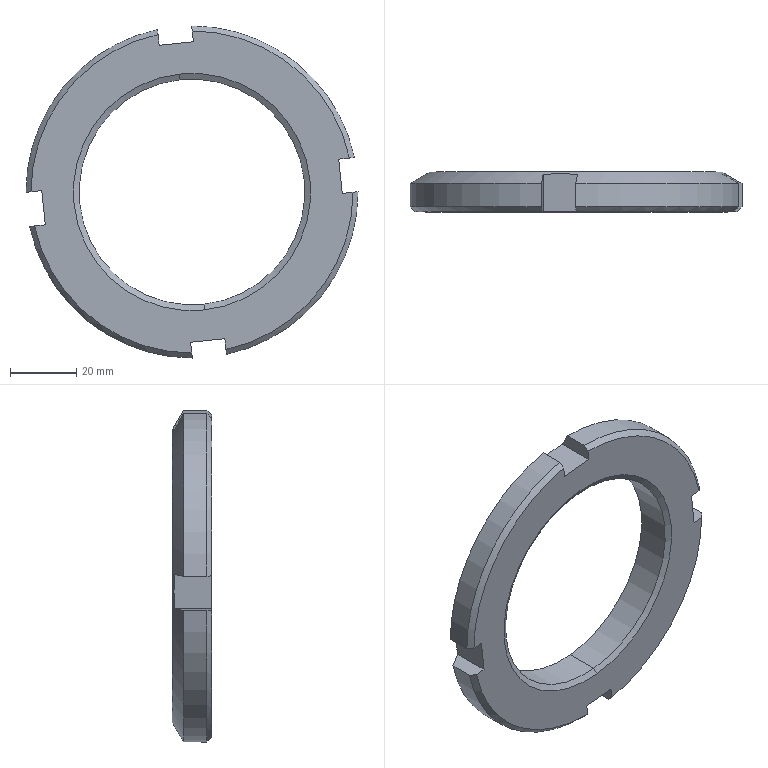Component | SolidWorks | LowerTensioningDeviceAssembly-1_GB_T812-1988[RoundNutM68_2]-1 | 1 solid | 30 faces | box 100 x 12 x 100 mm | volume 44820 mm3 | plane 14 | cone 10 | cylinder 6 | commonest cylinder face diameters 100 x4 68 x2
STEP:
#1=COLOUR_RGB('',0.7922,0.8196,0.9333);
#2=FILL_AREA_STYLE_COLOUR('',#1);
#3=FILL_AREA_STYLE('',(#2));
#4=SURFACE_STYLE_FILL_AREA(#3);
#5=SURFACE_SIDE_STYLE('',(#4));
#6=SURFACE_STYLE_USAGE(.BOTH.,#5);
#7=PRESENTATION_STYLE_ASSIGNMENT((#6));
#8=CARTESIAN_POINT('',(-0.1409,6.654,0.03981));
#9=VERTEX_POINT('',#8);
#10=CARTESIAN_POINT('',(0.1409,6.654,-2.622));
#11=VERTEX_POINT('',#10);
#12=CARTESIAN_POINT('',(-0.,6.654,-1.291));
#13=DIRECTION('',(-0.,-1.,-0.));
#14=DIRECTION('',(0.1053,0.,-0.9944));
#15=AXIS2_PLACEMENT_3D('',#12,#13,#14);
#16=CIRCLE('',#15,1.339);
#17=EDGE_CURVE('',#9,#11,#16,.T.);
#18=ORIENTED_EDGE('',*,*,#17,.F.);
#19=CARTESIAN_POINT('',(-0.1481,6.614,0.1076));
#20=VERTEX_POINT('',#19);
#21=CARTESIAN_POINT('',(-0.1409,6.654,0.03981));
#22=DIRECTION('',(-0.09115,-0.5,0.8612));
#23=VECTOR('',#22,39.37);
#24=LINE('',#21,#23);
#25=EDGE_CURVE('',#9,#20,#24,.T.);
#26=ORIENTED_EDGE('',*,*,#25,.T.);
#27=CARTESIAN_POINT('',(0.1481,6.614,-2.69));
#28=VERTEX_POINT('',#27);
#29=CARTESIAN_POINT('',(-0.,6.614,-1.291));
#30=DIRECTION('',(0.,1.,0.));
#31=DIRECTION('',(0.1053,0.,-0.9944));
#32=AXIS2_PLACEMENT_3D('',#29,#30,#31);
#33=CIRCLE('',#32,1.407);
#34=EDGE_CURVE('',#28,#20,#33,.T.);
#35=ORIENTED_EDGE('',*,*,#34,.F.);
#36=CARTESIAN_POINT('',(0.1409,6.654,-2.622));
#37=DIRECTION('',(0.09115,-0.5,-0.8612));
#38=VECTOR('',#37,39.37);
#39=LINE('',#36,#38);
#40=EDGE_CURVE('',#11,#28,#39,.T.);
#41=ORIENTED_EDGE('',*,*,#40,.F.);
#42=EDGE_LOOP('',(#18,#26,#35,#41));
#43=FACE_OUTER_BOUND('',#42,.T.);
#44=CARTESIAN_POINT('',(-0.,6.654,-1.291));
#45=DIRECTION('',(-0.,-1.,-0.));
#46=DIRECTION('',(0.1053,0.,-0.9944));
#47=AXIS2_PLACEMENT_3D('',#44,#45,#46);
#48=CONICAL_SURFACE('',#47,1.339,1.047);
#49=ADVANCED_FACE('',(#43),#48,.F.);
#50=CARTESIAN_POINT('',(0.1409,7.047,-2.622));
#51=VERTEX_POINT('',#50);
#52=CARTESIAN_POINT('',(-0.1409,7.047,0.03981));
#53=VERTEX_POINT('',#52);
#54=CARTESIAN_POINT('',(-0.,7.047,-1.291));
#55=DIRECTION('',(0.,1.,0.));
#56=DIRECTION('',(0.1053,0.,-0.9944));
#57=AXIS2_PLACEMENT_3D('',#54,#55,#56);
#58=CIRCLE('',#57,1.339);
#59=EDGE_CURVE('',#51,#53,#58,.T.);
#60=ORIENTED_EDGE('',*,*,#59,.F.);
#61=CARTESIAN_POINT('',(0.1481,7.087,-2.69));
#62=VERTEX_POINT('',#61);
#63=CARTESIAN_POINT('',(0.1481,7.087,-2.69));
#64=DIRECTION('',(0.09115,0.5,-0.8612));
#65=VECTOR('',#64,39.37);
#66=LINE('',#63,#65);
#67=EDGE_CURVE('',#51,#62,#66,.T.);
#68=ORIENTED_EDGE('',*,*,#67,.T.);
#69=CARTESIAN_POINT('',(-0.1481,7.087,0.1076));
#70=VERTEX_POINT('',#69);
#71=CARTESIAN_POINT('',(-0.,7.087,-1.291));
#72=DIRECTION('',(-0.,-1.,-0.));
#73=DIRECTION('',(0.1053,0.,-0.9944));
#74=AXIS2_PLACEMENT_3D('',#71,#72,#73);
#75=CIRCLE('',#74,1.407);
#76=EDGE_CURVE('',#70,#62,#75,.T.);
#77=ORIENTED_EDGE('',*,*,#76,.F.);
#78=CARTESIAN_POINT('',(-0.1481,7.087,0.1076));
#79=DIRECTION('',(-0.09115,0.5,0.8612));
#80=VECTOR('',#79,39.37);
#81=LINE('',#78,#80);
#82=EDGE_CURVE('',#53,#70,#81,.T.);
#83=ORIENTED_EDGE('',*,*,#82,.F.);
#84=EDGE_LOOP('',(#60,#68,#77,#83));
#85=FACE_OUTER_BOUND('',#84,.T.);
#86=CARTESIAN_POINT('',(-0.,7.087,-1.291));
#87=DIRECTION('',(0.,1.,0.));
#88=DIRECTION('',(-0.1053,-0.,0.9944));
#89=AXIS2_PLACEMENT_3D('',#86,#87,#88);
#90=CONICAL_SURFACE('',#89,1.407,1.047);
#91=ADVANCED_FACE('',(#85),#90,.F.);
#92=CARTESIAN_POINT('',(-0.1823,7.087,0.4313));
#93=VERTEX_POINT('',#92);
#94=CARTESIAN_POINT('',(0.1823,7.087,-3.014));
#95=VERTEX_POINT('',#94);
#96=CARTESIAN_POINT('',(-0.,7.087,-1.291));
#97=DIRECTION('',(0.,1.,0.));
#98=DIRECTION('',(0.1053,0.,-0.9944));
#99=AXIS2_PLACEMENT_3D('',#96,#97,#98);
#100=CIRCLE('',#99,1.732);
#101=EDGE_CURVE('',#93,#95,#100,.T.);
#102=ORIENTED_EDGE('',*,*,#101,.F.);
#103=CARTESIAN_POINT('',(-0.1864,7.064,0.4697));
#104=VERTEX_POINT('',#103);
#105=CARTESIAN_POINT('',(-0.2072,6.95,0.6662));
#106=DIRECTION('',(-0.09115,-0.5,0.8612));
#107=VECTOR('',#106,39.37);
#108=LINE('',#105,#107);
#109=EDGE_CURVE('',#93,#104,#108,.T.);
#110=ORIENTED_EDGE('',*,*,#109,.T.);
#111=CARTESIAN_POINT('',(0.01641,7.058,0.4912));
#112=VERTEX_POINT('',#111);
#113=CARTESIAN_POINT('',(0.01641,7.058,0.4912));
#114=CARTESIAN_POINT('',(-0.051,7.062,0.4841));
#115=CARTESIAN_POINT('',(-0.1186,7.064,0.4769));
#116=CARTESIAN_POINT('',(-0.1864,7.064,0.4697));
#117=B_SPLINE_CURVE_WITH_KNOTS('',3,(#113,#114,#115,#116),.UNSPECIFIED.,.F.,.F.,(4,4),(0.01245,0.01763),.UNSPECIFIED.);
#118=EDGE_CURVE('',#112,#104,#117,.T.);
#119=ORIENTED_EDGE('',*,*,#118,.F.);
#120=CARTESIAN_POINT('',(-0.003271,6.95,0.6772));
#121=VERTEX_POINT('',#120);
#122=CARTESIAN_POINT('',(-0.003271,6.95,0.6772));
#123=CARTESIAN_POINT('',(-0.002137,6.956,0.6665));
#124=CARTESIAN_POINT('',(-0.001004,6.963,0.6557));
#125=CARTESIAN_POINT('',(0.0001294,6.969,0.645));
#126=CARTESIAN_POINT('',(0.005556,6.998,0.5938));
#127=CARTESIAN_POINT('',(0.01098,7.028,0.5425));
#128=CARTESIAN_POINT('',(0.01641,7.058,0.4912));
#129=B_SPLINE_CURVE_WITH_KNOTS('',3,(#122,#123,#124,#125,#126,#127,#128),.UNSPECIFIED.,.F.,.F.,(4,3,4),(0.01027,0.01122,0.01575),.UNSPECIFIED.);
#130=EDGE_CURVE('',#121,#112,#129,.T.);
#131=ORIENTED_EDGE('',*,*,#130,.F.);
#132=CARTESIAN_POINT('',(1.926,6.95,-0.8825));
#133=VERTEX_POINT('',#132);
#134=CARTESIAN_POINT('',(-0.,6.95,-1.291));
#135=DIRECTION('',(-0.,-1.,-0.));
#136=DIRECTION('',(0.1053,0.,-0.9944));
#137=AXIS2_PLACEMENT_3D('',#134,#135,#136);
#138=CIRCLE('',#137,1.969);
#139=EDGE_CURVE('',#133,#121,#138,.T.);
#140=ORIENTED_EDGE('',*,*,#139,.F.);
#141=CARTESIAN_POINT('',(1.74,7.058,-0.9021));
#142=VERTEX_POINT('',#141);
#143=CARTESIAN_POINT('',(1.74,7.058,-0.9021));
#144=CARTESIAN_POINT('',(1.802,7.022,-0.8956));
#145=CARTESIAN_POINT('',(1.864,6.986,-0.889));
#146=CARTESIAN_POINT('',(1.926,6.95,-0.8825));
#147=B_SPLINE_CURVE_WITH_KNOTS('',3,(#143,#144,#145,#146),.UNSPECIFIED.,.F.,.F.,(4,4),(0.01064,0.01612),.UNSPECIFIED.);
#148=EDGE_CURVE('',#142,#133,#147,.T.);
#149=ORIENTED_EDGE('',*,*,#148,.F.);
#150=CARTESIAN_POINT('',(1.783,7.058,-1.308));
#151=VERTEX_POINT('',#150);
#152=CARTESIAN_POINT('',(1.783,7.058,-1.308));
#153=CARTESIAN_POINT('',(1.775,7.062,-1.241));
#154=CARTESIAN_POINT('',(1.768,7.064,-1.173));
#155=CARTESIAN_POINT('',(1.758,7.064,-1.072));
#156=CARTESIAN_POINT('',(1.754,7.064,-1.038));
#157=CARTESIAN_POINT('',(1.747,7.062,-0.97));
#158=CARTESIAN_POINT('',(1.743,7.06,-0.936));
#159=CARTESIAN_POINT('',(1.74,7.058,-0.9021));
#160=B_SPLINE_CURVE_WITH_KNOTS('',3,(#152,#153,#154,#155,#156,#157,#158,#159),.UNSPECIFIED.,.F.,.F.,(4,2,2,4),(0.01245,0.01761,0.02019,0.02278),.UNSPECIFIED.);
#161=EDGE_CURVE('',#151,#142,#160,.T.);
#162=ORIENTED_EDGE('',*,*,#161,.F.);
#163=CARTESIAN_POINT('',(1.969,6.95,-1.288));
#164=VERTEX_POINT('',#163);
#165=CARTESIAN_POINT('',(1.969,6.95,-1.288));
#166=CARTESIAN_POINT('',(1.907,6.986,-1.295));
#167=CARTESIAN_POINT('',(1.845,7.022,-1.301));
#168=CARTESIAN_POINT('',(1.783,7.058,-1.308));
#169=B_SPLINE_CURVE_WITH_KNOTS('',3,(#165,#166,#167,#168),.UNSPECIFIED.,.F.,.F.,(4,4),(0.006321,0.0118),.UNSPECIFIED.);
#170=EDGE_CURVE('',#164,#151,#169,.T.);
#171=ORIENTED_EDGE('',*,*,#170,.F.);
#172=CARTESIAN_POINT('',(0.4089,6.95,-3.217));
#173=VERTEX_POINT('',#172);
#174=CARTESIAN_POINT('',(-0.,6.95,-1.291));
#175=DIRECTION('',(-0.,-1.,-0.));
#176=DIRECTION('',(0.1053,0.,-0.9944));
#177=AXIS2_PLACEMENT_3D('',#174,#175,#176);
#178=CIRCLE('',#177,1.969);
#179=EDGE_CURVE('',#173,#164,#178,.T.);
#180=ORIENTED_EDGE('',*,*,#179,.F.);
#181=CARTESIAN_POINT('',(0.3892,7.058,-3.031));
#182=VERTEX_POINT('',#181);
#183=CARTESIAN_POINT('',(0.3892,7.058,-3.031));
#184=CARTESIAN_POINT('',(0.3958,7.022,-3.093));
#185=CARTESIAN_POINT('',(0.4023,6.986,-3.155));
#186=CARTESIAN_POINT('',(0.4089,6.95,-3.217));
#187=B_SPLINE_CURVE_WITH_KNOTS('',3,(#183,#184,#185,#186),.UNSPECIFIED.,.F.,.F.,(4,4),(0.01064,0.01612),.UNSPECIFIED.);
#188=EDGE_CURVE('',#182,#173,#187,.T.);
#189=ORIENTED_EDGE('',*,*,#188,.F.);
#190=CARTESIAN_POINT('',(0.1864,7.064,-3.052));
#191=VERTEX_POINT('',#190);
#192=CARTESIAN_POINT('',(0.1864,7.064,-3.052));
#193=CARTESIAN_POINT('',(0.2542,7.064,-3.045));
#194=CARTESIAN_POINT('',(0.3218,7.062,-3.038));
#195=CARTESIAN_POINT('',(0.3892,7.058,-3.031));
#196=B_SPLINE_CURVE_WITH_KNOTS('',3,(#192,#193,#194,#195),.UNSPECIFIED.,.F.,.F.,(4,4),(0.02543,0.03061),.UNSPECIFIED.);
#197=EDGE_CURVE('',#191,#182,#196,.T.);
#198=ORIENTED_EDGE('',*,*,#197,.F.);
#199=CARTESIAN_POINT('',(0.2072,6.95,-3.249));
#200=DIRECTION('',(0.09115,-0.5,-0.8612));
#201=VECTOR('',#200,39.37);
#202=LINE('',#199,#201);
#203=EDGE_CURVE('',#95,#191,#202,.T.);
#204=ORIENTED_EDGE('',*,*,#203,.F.);
#205=EDGE_LOOP('',(#102,#110,#119,#131,#140,#149,#162,#171,#180,#189,#198,#204));
#206=FACE_OUTER_BOUND('',#205,.T.);
#207=CARTESIAN_POINT('',(-0.,6.95,-1.291));
#208=DIRECTION('',(-0.,-1.,-0.));
#209=DIRECTION('',(0.1053,0.,-0.9944));
#210=AXIS2_PLACEMENT_3D('',#207,#208,#209);
#211=CONICAL_SURFACE('',#210,1.969,1.047);
#212=ADVANCED_FACE('',(#206),#211,.T.);
#213=ORIENTED_EDGE('',*,*,#17,.T.);
#214=CARTESIAN_POINT('',(0.1409,6.614,-2.622));
#215=DIRECTION('',(0.,1.,0.));
#216=VECTOR('',#215,39.37);
#217=LINE('',#214,#216);
#218=EDGE_CURVE('',#11,#51,#217,.T.);
#219=ORIENTED_EDGE('',*,*,#218,.T.);
#220=ORIENTED_EDGE('',*,*,#59,.T.);
#221=CARTESIAN_POINT('',(-0.1409,6.614,0.03981));
#222=DIRECTION('',(0.,1.,0.));
#223=VECTOR('',#222,39.37);
#224=LINE('',#221,#223);
#225=EDGE_CURVE('',#9,#53,#224,.T.);
#226=ORIENTED_EDGE('',*,*,#225,.F.);
#227=EDGE_LOOP('',(#213,#219,#220,#226));
#228=FACE_OUTER_BOUND('',#227,.T.);
#229=CARTESIAN_POINT('',(-0.,6.614,-1.291));
#230=DIRECTION('',(0.,1.,0.));
#231=DIRECTION('',(-0.1053,-0.,0.9944));
#232=AXIS2_PLACEMENT_3D('',#229,#230,#231);
#233=CYLINDRICAL_SURFACE('',#232,1.339);
#234=ADVANCED_FACE('',(#228),#233,.F.);
#235=CARTESIAN_POINT('',(1.969,6.673,-1.288));
#236=VERTEX_POINT('',#235);
#237=CARTESIAN_POINT('',(0.4089,6.673,-3.217));
#238=VERTEX_POINT('',#237);
#239=CARTESIAN_POINT('',(-0.,6.673,-1.291));
#240=DIRECTION('',(0.,1.,0.));
#241=DIRECTION('',(0.1053,0.,-0.9944));
#242=AXIS2_PLACEMENT_3D('',#239,#240,#241);
#243=CIRCLE('',#242,1.969);
#244=EDGE_CURVE('',#236,#238,#243,.T.);
#245=ORIENTED_EDGE('',*,*,#244,.T.);
#246=CARTESIAN_POINT('',(0.4089,7.087,-3.217));
#247=DIRECTION('',(-0.,-1.,-0.));
#248=VECTOR('',#247,39.37);
#249=LINE('',#246,#248);
#250=EDGE_CURVE('',#173,#238,#249,.T.);
#251=ORIENTED_EDGE('',*,*,#250,.F.);
#252=ORIENTED_EDGE('',*,*,#179,.T.);
#253=CARTESIAN_POINT('',(1.969,7.087,-1.288));
#254=DIRECTION('',(-0.,-1.,-0.));
#255=VECTOR('',#254,39.37);
#256=LINE('',#253,#255);
#257=EDGE_CURVE('',#164,#236,#256,.T.);
#258=ORIENTED_EDGE('',*,*,#257,.T.);
#259=EDGE_LOOP('',(#245,#251,#252,#258));
#260=FACE_OUTER_BOUND('',#259,.T.);
#261=CARTESIAN_POINT('',(-0.,6.614,-1.291));
#262=DIRECTION('',(0.,1.,0.));
#263=DIRECTION('',(-0.1053,-0.,0.9944));
#264=AXIS2_PLACEMENT_3D('',#261,#262,#263);
#265=CYLINDRICAL_SURFACE('',#264,1.969);
#266=ADVANCED_FACE('',(#260),#265,.T.);
#267=CARTESIAN_POINT('',(0.4026,6.614,-3.158));
#268=VERTEX_POINT('',#267);
#269=CARTESIAN_POINT('',(0.4089,6.673,-3.217));
#270=CARTESIAN_POINT('',(0.4071,6.657,-3.2));
#271=CARTESIAN_POINT('',(0.4054,6.64,-3.184));
#272=CARTESIAN_POINT('',(0.4036,6.623,-3.167));
#273=CARTESIAN_POINT('',(0.4033,6.62,-3.164));
#274=CARTESIAN_POINT('',(0.403,6.617,-3.161));
#275=CARTESIAN_POINT('',(0.4026,6.614,-3.158));
#276=B_SPLINE_CURVE_WITH_KNOTS('',3,(#269,#270,#271,#272,#273,#274,#275),.UNSPECIFIED.,.F.,.F.,(4,3,4),(0.00787,0.009662,0.009997),.UNSPECIFIED.);
#277=EDGE_CURVE('',#238,#268,#276,.T.);
#278=ORIENTED_EDGE('',*,*,#277,.F.);
#279=ORIENTED_EDGE('',*,*,#244,.F.);
#280=CARTESIAN_POINT('',(1.909,6.614,-1.294));
#281=VERTEX_POINT('',#280);
#282=CARTESIAN_POINT('',(1.909,6.614,-1.294));
#283=CARTESIAN_POINT('',(1.913,6.617,-1.294));
#284=CARTESIAN_POINT('',(1.916,6.62,-1.294));
#285=CARTESIAN_POINT('',(1.919,6.623,-1.293));
#286=CARTESIAN_POINT('',(1.935,6.64,-1.292));
#287=CARTESIAN_POINT('',(1.952,6.657,-1.29));
#288=CARTESIAN_POINT('',(1.969,6.673,-1.288));
#289=B_SPLINE_CURVE_WITH_KNOTS('',3,(#282,#283,#284,#285,#286,#287,#288),.UNSPECIFIED.,.F.,.F.,(4,3,4),(0.009327,0.009662,0.01145),.UNSPECIFIED.);
#290=EDGE_CURVE('',#281,#236,#289,.T.);
#291=ORIENTED_EDGE('',*,*,#290,.F.);
#292=CARTESIAN_POINT('',(-0.,6.614,-1.291));
#293=DIRECTION('',(-0.,-1.,-0.));
#294=DIRECTION('',(0.1053,0.,-0.9944));
#295=AXIS2_PLACEMENT_3D('',#292,#293,#294);
#296=CIRCLE('',#295,1.909);
#297=EDGE_CURVE('',#268,#281,#296,.T.);
#298=ORIENTED_EDGE('',*,*,#297,.F.);
#299=EDGE_LOOP('',(#278,#279,#291,#298));
#300=FACE_OUTER_BOUND('',#299,.T.);
#301=CARTESIAN_POINT('',(-0.,6.614,-1.291));
#302=DIRECTION('',(0.,1.,0.));
#303=DIRECTION('',(-0.1053,-0.,0.9944));
#304=AXIS2_PLACEMENT_3D('',#301,#302,#303);
#305=CONICAL_SURFACE('',#304,1.909,0.7854);
#306=ADVANCED_FACE('',(#300),#305,.T.);
#307=CARTESIAN_POINT('',(-0.003271,6.673,0.6772));
#308=VERTEX_POINT('',#307);
#309=CARTESIAN_POINT('',(1.926,6.673,-0.8825));
#310=VERTEX_POINT('',#309);
#311=CARTESIAN_POINT('',(-0.,6.673,-1.291));
#312=DIRECTION('',(0.,1.,0.));
#313=DIRECTION('',(0.1053,0.,-0.9944));
#314=AXIS2_PLACEMENT_3D('',#311,#312,#313);
#315=CIRCLE('',#314,1.969);
#316=EDGE_CURVE('',#308,#310,#315,.T.);
#317=ORIENTED_EDGE('',*,*,#316,.T.);
#318=CARTESIAN_POINT('',(1.926,7.087,-0.8825));
#319=DIRECTION('',(-0.,-1.,-0.));
#320=VECTOR('',#319,39.37);
#321=LINE('',#318,#320);
#322=EDGE_CURVE('',#133,#310,#321,.T.);
#323=ORIENTED_EDGE('',*,*,#322,.F.);
#324=ORIENTED_EDGE('',*,*,#139,.T.);
#325=CARTESIAN_POINT('',(-0.003271,7.087,0.6772));
#326=DIRECTION('',(-0.,-1.,-0.));
#327=VECTOR('',#326,39.37);
#328=LINE('',#325,#327);
#329=EDGE_CURVE('',#121,#308,#328,.T.);
#330=ORIENTED_EDGE('',*,*,#329,.T.);
#331=EDGE_LOOP('',(#317,#323,#324,#330));
#332=FACE_OUTER_BOUND('',#331,.T.);
#333=CARTESIAN_POINT('',(-0.,6.614,-1.291));
#334=DIRECTION('',(0.,1.,0.));
#335=DIRECTION('',(-0.1053,-0.,0.9944));
#336=AXIS2_PLACEMENT_3D('',#333,#334,#335);
#337=CYLINDRICAL_SURFACE('',#336,1.969);
#338=ADVANCED_FACE('',(#332),#337,.T.);
#339=CARTESIAN_POINT('',(1.867,6.614,-0.8887));
#340=VERTEX_POINT('',#339);
#341=CARTESIAN_POINT('',(1.926,6.673,-0.8825));
#342=CARTESIAN_POINT('',(1.909,6.657,-0.8842));
#343=CARTESIAN_POINT('',(1.892,6.64,-0.886));
#344=CARTESIAN_POINT('',(1.876,6.623,-0.8877));
#345=CARTESIAN_POINT('',(1.873,6.62,-0.8881));
#346=CARTESIAN_POINT('',(1.87,6.617,-0.8884));
#347=CARTESIAN_POINT('',(1.867,6.614,-0.8887));
#348=B_SPLINE_CURVE_WITH_KNOTS('',3,(#341,#342,#343,#344,#345,#346,#347),.UNSPECIFIED.,.F.,.F.,(4,3,4),(0.00787,0.009662,0.009997),.UNSPECIFIED.);
#349=EDGE_CURVE('',#310,#340,#348,.T.);
#350=ORIENTED_EDGE('',*,*,#349,.F.);
#351=ORIENTED_EDGE('',*,*,#316,.F.);
#352=CARTESIAN_POINT('',(0.00298,6.614,0.6181));
#353=VERTEX_POINT('',#352);
#354=CARTESIAN_POINT('',(0.00298,6.614,0.6181));
#355=CARTESIAN_POINT('',(0.001827,6.625,0.629));
#356=CARTESIAN_POINT('',(0.0006734,6.636,0.6399));
#357=CARTESIAN_POINT('',(-0.0004797,6.647,0.6508));
#358=CARTESIAN_POINT('',(-0.00141,6.656,0.6596));
#359=CARTESIAN_POINT('',(-0.00234,6.664,0.6684));
#360=CARTESIAN_POINT('',(-0.003271,6.673,0.6772));
#361=B_SPLINE_CURVE_WITH_KNOTS('',3,(#354,#355,#356,#357,#358,#359,#360),.UNSPECIFIED.,.F.,.F.,(4,3,4),(0.008485,0.009662,0.01061),.UNSPECIFIED.);
#362=EDGE_CURVE('',#353,#308,#361,.T.);
#363=ORIENTED_EDGE('',*,*,#362,.F.);
#364=CARTESIAN_POINT('',(-0.,6.614,-1.291));
#365=DIRECTION('',(-0.,-1.,-0.));
#366=DIRECTION('',(0.1053,0.,-0.9944));
#367=AXIS2_PLACEMENT_3D('',#364,#365,#366);
#368=CIRCLE('',#367,1.909);
#369=EDGE_CURVE('',#340,#353,#368,.T.);
#370=ORIENTED_EDGE('',*,*,#369,.F.);
#371=EDGE_LOOP('',(#350,#351,#363,#370));
#372=FACE_OUTER_BOUND('',#371,.T.);
#373=CARTESIAN_POINT('',(-0.,6.614,-1.291));
#374=DIRECTION('',(0.,1.,0.));
#375=DIRECTION('',(-0.1053,-0.,0.9944));
#376=AXIS2_PLACEMENT_3D('',#373,#374,#375);
#377=CONICAL_SURFACE('',#376,1.909,0.7854);
#378=ADVANCED_FACE('',(#372),#377,.T.);
#379=CARTESIAN_POINT('',(-1.969,6.673,-1.295));
#380=VERTEX_POINT('',#379);
#381=CARTESIAN_POINT('',(-0.4089,6.673,0.6342));
#382=VERTEX_POINT('',#381);
#383=CARTESIAN_POINT('',(-0.,6.673,-1.291));
#384=DIRECTION('',(0.,1.,0.));
#385=DIRECTION('',(0.1053,0.,-0.9944));
#386=AXIS2_PLACEMENT_3D('',#383,#384,#385);
#387=CIRCLE('',#386,1.969);
#388=EDGE_CURVE('',#380,#382,#387,.T.);
#389=ORIENTED_EDGE('',*,*,#388,.T.);
#390=CARTESIAN_POINT('',(-0.4089,6.95,0.6342));
#391=VERTEX_POINT('',#390);
#392=CARTESIAN_POINT('',(-0.4089,7.087,0.6342));
#393=DIRECTION('',(-0.,-1.,-0.));
#394=VECTOR('',#393,39.37);
#395=LINE('',#392,#394);
#396=EDGE_CURVE('',#391,#382,#395,.T.);
#397=ORIENTED_EDGE('',*,*,#396,.F.);
#398=CARTESIAN_POINT('',(-1.969,6.95,-1.295));
#399=VERTEX_POINT('',#398);
#400=CARTESIAN_POINT('',(-0.,6.95,-1.291));
#401=DIRECTION('',(-0.,-1.,-0.));
#402=DIRECTION('',(0.1053,0.,-0.9944));
#403=AXIS2_PLACEMENT_3D('',#400,#401,#402);
#404=CIRCLE('',#403,1.969);
#405=EDGE_CURVE('',#391,#399,#404,.T.);
#406=ORIENTED_EDGE('',*,*,#405,.T.);
#407=CARTESIAN_POINT('',(-1.969,7.087,-1.295));
#408=DIRECTION('',(-0.,-1.,-0.));
#409=VECTOR('',#408,39.37);
#410=LINE('',#407,#409);
#411=EDGE_CURVE('',#399,#380,#410,.T.);
#412=ORIENTED_EDGE('',*,*,#411,.T.);
#413=EDGE_LOOP('',(#389,#397,#406,#412));
#414=FACE_OUTER_BOUND('',#413,.T.);
#415=CARTESIAN_POINT('',(-0.,6.614,-1.291));
#416=DIRECTION('',(0.,1.,0.));
#417=DIRECTION('',(-0.1053,-0.,0.9944));
#418=AXIS2_PLACEMENT_3D('',#415,#416,#417);
#419=CYLINDRICAL_SURFACE('',#418,1.969);
#420=ADVANCED_FACE('',(#414),#419,.T.);
#421=CARTESIAN_POINT('',(-0.4026,6.614,0.5752));
#422=VERTEX_POINT('',#421);
#423=CARTESIAN_POINT('',(-0.4089,6.673,0.6342));
#424=CARTESIAN_POINT('',(-0.4079,6.664,0.6254));
#425=CARTESIAN_POINT('',(-0.407,6.656,0.6167));
#426=CARTESIAN_POINT('',(-0.4061,6.647,0.6079));
#427=CARTESIAN_POINT('',(-0.4049,6.636,0.597));
#428=CARTESIAN_POINT('',(-0.4038,6.625,0.5861));
#429=CARTESIAN_POINT('',(-0.4026,6.614,0.5752));
#430=B_SPLINE_CURVE_WITH_KNOTS('',3,(#423,#424,#425,#426,#427,#428,#429),.UNSPECIFIED.,.F.,.F.,(4,3,4),(0.008712,0.009662,0.01084),.UNSPECIFIED.);
#431=EDGE_CURVE('',#382,#422,#430,.T.);
#432=ORIENTED_EDGE('',*,*,#431,.F.);
#433=ORIENTED_EDGE('',*,*,#388,.F.);
#434=CARTESIAN_POINT('',(-1.909,6.614,-1.288));
#435=VERTEX_POINT('',#434);
#436=CARTESIAN_POINT('',(-1.909,6.614,-1.288));
#437=CARTESIAN_POINT('',(-1.92,6.625,-1.29));
#438=CARTESIAN_POINT('',(-1.931,6.636,-1.291));
#439=CARTESIAN_POINT('',(-1.942,6.647,-1.292));
#440=CARTESIAN_POINT('',(-1.951,6.656,-1.293));
#441=CARTESIAN_POINT('',(-1.96,6.664,-1.294));
#442=CARTESIAN_POINT('',(-1.969,6.673,-1.295));
#443=B_SPLINE_CURVE_WITH_KNOTS('',3,(#436,#437,#438,#439,#440,#441,#442),.UNSPECIFIED.,.F.,.F.,(4,3,4),(0.008485,0.009662,0.01061),.UNSPECIFIED.);
#444=EDGE_CURVE('',#435,#380,#443,.T.);
#445=ORIENTED_EDGE('',*,*,#444,.F.);
#446=CARTESIAN_POINT('',(-0.,6.614,-1.291));
#447=DIRECTION('',(-0.,-1.,-0.));
#448=DIRECTION('',(0.1053,0.,-0.9944));
#449=AXIS2_PLACEMENT_3D('',#446,#447,#448);
#450=CIRCLE('',#449,1.909);
#451=EDGE_CURVE('',#422,#435,#450,.T.);
#452=ORIENTED_EDGE('',*,*,#451,.F.);
#453=EDGE_LOOP('',(#432,#433,#445,#452));
#454=FACE_OUTER_BOUND('',#453,.T.);
#455=CARTESIAN_POINT('',(-0.,6.614,-1.291));
#456=DIRECTION('',(0.,1.,0.));
#457=DIRECTION('',(-0.1053,-0.,0.9944));
#458=AXIS2_PLACEMENT_3D('',#455,#456,#457);
#459=CONICAL_SURFACE('',#458,1.909,0.7854);
#460=ADVANCED_FACE('',(#454),#459,.T.);
#461=ORIENTED_EDGE('',*,*,#34,.T.);
#462=CARTESIAN_POINT('',(-0.,6.614,-1.291));
#463=DIRECTION('',(0.,1.,0.));
#464=DIRECTION('',(0.1053,0.,-0.9944));
#465=AXIS2_PLACEMENT_3D('',#462,#463,#464);
#466=CIRCLE('',#465,1.407);
#467=EDGE_CURVE('',#20,#28,#466,.T.);
#468=ORIENTED_EDGE('',*,*,#467,.T.);
#469=EDGE_LOOP('',(#461,#468));
#470=FACE_BOUND('',#469,.T.);
#471=CARTESIAN_POINT('',(0.3892,6.614,-3.031));
#472=VERTEX_POINT('',#471);
#473=CARTESIAN_POINT('',(0.3892,6.614,-3.031));
#474=DIRECTION('',(-0.1053,-0.,0.9944));
#475=VECTOR('',#474,39.37);
#476=LINE('',#473,#475);
#477=EDGE_CURVE('',#268,#472,#476,.T.);
#478=ORIENTED_EDGE('',*,*,#477,.F.);
#479=ORIENTED_EDGE('',*,*,#297,.T.);
#480=CARTESIAN_POINT('',(1.783,6.614,-1.308));
#481=VERTEX_POINT('',#480);
#482=CARTESIAN_POINT('',(1.783,6.614,-1.308));
#483=DIRECTION('',(0.9944,-0.,0.1053));
#484=VECTOR('',#483,39.37);
#485=LINE('',#482,#484);
#486=EDGE_CURVE('',#481,#281,#485,.T.);
#487=ORIENTED_EDGE('',*,*,#486,.F.);
#488=CARTESIAN_POINT('',(1.74,6.614,-0.9021));
#489=VERTEX_POINT('',#488);
#490=CARTESIAN_POINT('',(1.783,6.614,-1.308));
#491=DIRECTION('',(0.1053,0.,-0.9944));
#492=VECTOR('',#491,39.37);
#493=LINE('',#490,#492);
#494=EDGE_CURVE('',#489,#481,#493,.T.);
#495=ORIENTED_EDGE('',*,*,#494,.F.);
#496=CARTESIAN_POINT('',(1.74,6.614,-0.9021));
#497=DIRECTION('',(-0.9944,0.,-0.1053));
#498=VECTOR('',#497,39.37);
#499=LINE('',#496,#498);
#500=EDGE_CURVE('',#340,#489,#499,.T.);
#501=ORIENTED_EDGE('',*,*,#500,.F.);
#502=ORIENTED_EDGE('',*,*,#369,.T.);
#503=CARTESIAN_POINT('',(0.01641,6.614,0.4912));
#504=VERTEX_POINT('',#503);
#505=CARTESIAN_POINT('',(0.01641,6.614,0.4912));
#506=DIRECTION('',(-0.1053,-0.,0.9944));
#507=VECTOR('',#506,39.37);
#508=LINE('',#505,#507);
#509=EDGE_CURVE('',#504,#353,#508,.T.);
#510=ORIENTED_EDGE('',*,*,#509,.F.);
#511=CARTESIAN_POINT('',(-0.3892,6.614,0.4483));
#512=VERTEX_POINT('',#511);
#513=CARTESIAN_POINT('',(0.01641,6.614,0.4912));
#514=DIRECTION('',(0.9944,-0.,0.1053));
#515=VECTOR('',#514,39.37);
#516=LINE('',#513,#515);
#517=EDGE_CURVE('',#512,#504,#516,.T.);
#518=ORIENTED_EDGE('',*,*,#517,.F.);
#519=CARTESIAN_POINT('',(-0.3892,6.614,0.4483));
#520=DIRECTION('',(0.1053,0.,-0.9944));
#521=VECTOR('',#520,39.37);
#522=LINE('',#519,#521);
#523=EDGE_CURVE('',#422,#512,#522,.T.);
#524=ORIENTED_EDGE('',*,*,#523,.F.);
#525=ORIENTED_EDGE('',*,*,#451,.T.);
#526=CARTESIAN_POINT('',(-1.783,6.614,-1.275));
#527=VERTEX_POINT('',#526);
#528=CARTESIAN_POINT('',(-1.783,6.614,-1.275));
#529=DIRECTION('',(-0.9944,0.,-0.1053));
#530=VECTOR('',#529,39.37);
#531=LINE('',#528,#530);
#532=EDGE_CURVE('',#527,#435,#531,.T.);
#533=ORIENTED_EDGE('',*,*,#532,.F.);
#534=CARTESIAN_POINT('',(-1.74,6.614,-1.681));
#535=VERTEX_POINT('',#534);
#536=CARTESIAN_POINT('',(-1.783,6.614,-1.275));
#537=DIRECTION('',(-0.1053,-0.,0.9944));
#538=VECTOR('',#537,39.37);
#539=LINE('',#536,#538);
#540=EDGE_CURVE('',#535,#527,#539,.T.);
#541=ORIENTED_EDGE('',*,*,#540,.F.);
#542=CARTESIAN_POINT('',(-1.867,6.614,-1.694));
#543=VERTEX_POINT('',#542);
#544=CARTESIAN_POINT('',(-1.74,6.614,-1.681));
#545=DIRECTION('',(0.9944,-0.,0.1053));
#546=VECTOR('',#545,39.37);
#547=LINE('',#544,#546);
#548=EDGE_CURVE('',#543,#535,#547,.T.);
#549=ORIENTED_EDGE('',*,*,#548,.F.);
#550=CARTESIAN_POINT('',(-0.00298,6.614,-3.201));
#551=VERTEX_POINT('',#550);
#552=CARTESIAN_POINT('',(-0.,6.614,-1.291));
#553=DIRECTION('',(-0.,-1.,-0.));
#554=DIRECTION('',(0.1053,0.,-0.9944));
#555=AXIS2_PLACEMENT_3D('',#552,#553,#554);
#556=CIRCLE('',#555,1.909);
#557=EDGE_CURVE('',#543,#551,#556,.T.);
#558=ORIENTED_EDGE('',*,*,#557,.T.);
#559=CARTESIAN_POINT('',(-0.01641,6.614,-3.074));
#560=VERTEX_POINT('',#559);
#561=CARTESIAN_POINT('',(-0.01641,6.614,-3.074));
#562=DIRECTION('',(0.1053,0.,-0.9944));
#563=VECTOR('',#562,39.37);
#564=LINE('',#561,#563);
#565=EDGE_CURVE('',#560,#551,#564,.T.);
#566=ORIENTED_EDGE('',*,*,#565,.F.);
#567=CARTESIAN_POINT('',(-0.01641,6.614,-3.074));
#568=DIRECTION('',(-0.9944,0.,-0.1053));
#569=VECTOR('',#568,39.37);
#570=LINE('',#567,#569);
#571=EDGE_CURVE('',#472,#560,#570,.T.);
#572=ORIENTED_EDGE('',*,*,#571,.F.);
#573=EDGE_LOOP('',(#478,#479,#487,#495,#501,#502,#510,#518,#524,#525,#533,#541,#549,#558,#566,#572));
#574=FACE_OUTER_BOUND('',#573,.T.);
#575=CARTESIAN_POINT('',(-0.,6.614,-1.291));
#576=DIRECTION('',(-0.,-1.,-0.));
#577=DIRECTION('',(0.1053,0.,-0.9944));
#578=AXIS2_PLACEMENT_3D('',#575,#576,#577);
#579=PLANE('',#578);
#580=ADVANCED_FACE('',(#470,#574),#579,.T.);
#581=ORIENTED_EDGE('',*,*,#76,.T.);
#582=CARTESIAN_POINT('',(-0.,7.087,-1.291));
#583=DIRECTION('',(-0.,-1.,-0.));
#584=DIRECTION('',(0.1053,0.,-0.9944));
#585=AXIS2_PLACEMENT_3D('',#582,#583,#584);
#586=CIRCLE('',#585,1.407);
#587=EDGE_CURVE('',#62,#70,#586,.T.);
#588=ORIENTED_EDGE('',*,*,#587,.T.);
#589=EDGE_LOOP('',(#581,#588));
#590=FACE_BOUND('',#589,.T.);
#591=CARTESIAN_POINT('',(-0.,7.087,-1.291));
#592=DIRECTION('',(0.,1.,0.));
#593=DIRECTION('',(0.1053,0.,-0.9944));
#594=AXIS2_PLACEMENT_3D('',#591,#592,#593);
#595=CIRCLE('',#594,1.732);
#596=EDGE_CURVE('',#95,#93,#595,.T.);
#597=ORIENTED_EDGE('',*,*,#596,.T.);
#598=ORIENTED_EDGE('',*,*,#101,.T.);
#599=EDGE_LOOP('',(#597,#598));
#600=FACE_OUTER_BOUND('',#599,.T.);
#601=CARTESIAN_POINT('',(-0.,7.087,-1.291));
#602=DIRECTION('',(-0.,-1.,-0.));
#603=DIRECTION('',(0.1053,0.,-0.9944));
#604=AXIS2_PLACEMENT_3D('',#601,#602,#603);
#605=PLANE('',#604);
#606=ADVANCED_FACE('',(#590,#600),#605,.F.);
#607=CARTESIAN_POINT('',(-1.926,6.95,-1.7));
#608=VERTEX_POINT('',#607);
#609=CARTESIAN_POINT('',(0.003271,6.95,-3.26));
#610=VERTEX_POINT('',#609);
#611=CARTESIAN_POINT('',(-0.,6.95,-1.291));
#612=DIRECTION('',(-0.,-1.,-0.));
#613=DIRECTION('',(0.1053,0.,-0.9944));
#614=AXIS2_PLACEMENT_3D('',#611,#612,#613);
#615=CIRCLE('',#614,1.969);
#616=EDGE_CURVE('',#608,#610,#615,.T.);
#617=ORIENTED_EDGE('',*,*,#616,.T.);
#618=CARTESIAN_POINT('',(0.003271,6.673,-3.26));
#619=VERTEX_POINT('',#618);
#620=CARTESIAN_POINT('',(0.003271,7.087,-3.26));
#621=DIRECTION('',(-0.,-1.,-0.));
#622=VECTOR('',#621,39.37);
#623=LINE('',#620,#622);
#624=EDGE_CURVE('',#610,#619,#623,.T.);
#625=ORIENTED_EDGE('',*,*,#624,.T.);
#626=CARTESIAN_POINT('',(-1.926,6.673,-1.7));
#627=VERTEX_POINT('',#626);
#628=CARTESIAN_POINT('',(-0.,6.673,-1.291));
#629=DIRECTION('',(0.,1.,0.));
#630=DIRECTION('',(0.1053,0.,-0.9944));
#631=AXIS2_PLACEMENT_3D('',#628,#629,#630);
#632=CIRCLE('',#631,1.969);
#633=EDGE_CURVE('',#619,#627,#632,.T.);
#634=ORIENTED_EDGE('',*,*,#633,.T.);
#635=CARTESIAN_POINT('',(-1.926,7.087,-1.7));
#636=DIRECTION('',(-0.,-1.,-0.));
#637=VECTOR('',#636,39.37);
#638=LINE('',#635,#637);
#639=EDGE_CURVE('',#608,#627,#638,.T.);
#640=ORIENTED_EDGE('',*,*,#639,.F.);
#641=EDGE_LOOP('',(#617,#625,#634,#640));
#642=FACE_OUTER_BOUND('',#641,.T.);
#643=CARTESIAN_POINT('',(-0.,6.614,-1.291));
#644=DIRECTION('',(0.,1.,0.));
#645=DIRECTION('',(-0.1053,-0.,0.9944));
#646=AXIS2_PLACEMENT_3D('',#643,#644,#645);
#647=CYLINDRICAL_SURFACE('',#646,1.969);
#648=ADVANCED_FACE('',(#642),#647,.T.);
#649=ORIENTED_EDGE('',*,*,#218,.F.);
#650=CARTESIAN_POINT('',(-0.,6.654,-1.291));
#651=DIRECTION('',(-0.,-1.,-0.));
#652=DIRECTION('',(0.1053,0.,-0.9944));
#653=AXIS2_PLACEMENT_3D('',#650,#651,#652);
#654=CIRCLE('',#653,1.339);
#655=EDGE_CURVE('',#11,#9,#654,.T.);
#656=ORIENTED_EDGE('',*,*,#655,.T.);
#657=ORIENTED_EDGE('',*,*,#225,.T.);
#658=CARTESIAN_POINT('',(-0.,7.047,-1.291));
#659=DIRECTION('',(0.,1.,0.));
#660=DIRECTION('',(0.1053,0.,-0.9944));
#661=AXIS2_PLACEMENT_3D('',#658,#659,#660);
#662=CIRCLE('',#661,1.339);
#663=EDGE_CURVE('',#53,#51,#662,.T.);
#664=ORIENTED_EDGE('',*,*,#663,.T.);
#665=EDGE_LOOP('',(#649,#656,#657,#664));
#666=FACE_OUTER_BOUND('',#665,.T.);
#667=CARTESIAN_POINT('',(-0.,6.614,-1.291));
#668=DIRECTION('',(0.,1.,0.));
#669=DIRECTION('',(-0.1053,-0.,0.9944));
#670=AXIS2_PLACEMENT_3D('',#667,#668,#669);
#671=CYLINDRICAL_SURFACE('',#670,1.339);
#672=ADVANCED_FACE('',(#666),#671,.F.);
#673=CARTESIAN_POINT('',(-0.00298,6.614,-3.201));
#674=CARTESIAN_POINT('',(-0.002651,6.617,-3.204));
#675=CARTESIAN_POINT('',(-0.002323,6.62,-3.207));
#676=CARTESIAN_POINT('',(-0.001995,6.623,-3.21));
#677=CARTESIAN_POINT('',(-0.0002395,6.64,-3.227));
#678=CARTESIAN_POINT('',(0.001516,6.657,-3.243));
#679=CARTESIAN_POINT('',(0.003271,6.673,-3.26));
#680=B_SPLINE_CURVE_WITH_KNOTS('',3,(#673,#674,#675,#676,#677,#678,#679),.UNSPECIFIED.,.F.,.F.,(4,3,4),(0.009327,0.009662,0.01145),.UNSPECIFIED.);
#681=EDGE_CURVE('',#551,#619,#680,.T.);
#682=ORIENTED_EDGE('',*,*,#681,.F.);
#683=ORIENTED_EDGE('',*,*,#557,.F.);
#684=CARTESIAN_POINT('',(-1.926,6.673,-1.7));
#685=CARTESIAN_POINT('',(-1.917,6.664,-1.699));
#686=CARTESIAN_POINT('',(-1.908,6.656,-1.698));
#687=CARTESIAN_POINT('',(-1.899,6.647,-1.697));
#688=CARTESIAN_POINT('',(-1.888,6.636,-1.696));
#689=CARTESIAN_POINT('',(-1.877,6.625,-1.695));
#690=CARTESIAN_POINT('',(-1.867,6.614,-1.694));
#691=B_SPLINE_CURVE_WITH_KNOTS('',3,(#684,#685,#686,#687,#688,#689,#690),.UNSPECIFIED.,.F.,.F.,(4,3,4),(0.008712,0.009662,0.01084),.UNSPECIFIED.);
#692=EDGE_CURVE('',#627,#543,#691,.T.);
#693=ORIENTED_EDGE('',*,*,#692,.F.);
#694=ORIENTED_EDGE('',*,*,#633,.F.);
#695=EDGE_LOOP('',(#682,#683,#693,#694));
#696=FACE_OUTER_BOUND('',#695,.T.);
#697=CARTESIAN_POINT('',(-0.,6.614,-1.291));
#698=DIRECTION('',(0.,1.,0.));
#699=DIRECTION('',(-0.1053,-0.,0.9944));
#700=AXIS2_PLACEMENT_3D('',#697,#698,#699);
#701=CONICAL_SURFACE('',#700,1.909,0.7854);
#702=ADVANCED_FACE('',(#696),#701,.T.);
#703=ORIENTED_EDGE('',*,*,#109,.F.);
#704=ORIENTED_EDGE('',*,*,#596,.F.);
#705=ORIENTED_EDGE('',*,*,#203,.T.);
#706=CARTESIAN_POINT('',(-0.01641,7.058,-3.074));
#707=VERTEX_POINT('',#706);
#708=CARTESIAN_POINT('',(-0.01641,7.058,-3.074));
#709=CARTESIAN_POINT('',(0.01736,7.06,-3.07));
#710=CARTESIAN_POINT('',(0.05126,7.061,-3.067));
#711=CARTESIAN_POINT('',(0.1189,7.064,-3.06));
#712=CARTESIAN_POINT('',(0.1527,7.064,-3.056));
#713=CARTESIAN_POINT('',(0.1864,7.064,-3.052));
#714=B_SPLINE_CURVE_WITH_KNOTS('',3,(#708,#709,#710,#711,#712,#713),.UNSPECIFIED.,.F.,.F.,(4,2,4),(0.02027,0.02285,0.02543),.UNSPECIFIED.);
#715=EDGE_CURVE('',#707,#191,#714,.T.);
#716=ORIENTED_EDGE('',*,*,#715,.F.);
#717=CARTESIAN_POINT('',(0.003271,6.95,-3.26));
#718=CARTESIAN_POINT('',(-0.00329,6.986,-3.198));
#719=CARTESIAN_POINT('',(-0.00985,7.022,-3.136));
#720=CARTESIAN_POINT('',(-0.01641,7.058,-3.074));
#721=B_SPLINE_CURVE_WITH_KNOTS('',3,(#717,#718,#719,#720),.UNSPECIFIED.,.F.,.F.,(4,4),(0.006321,0.0118),.UNSPECIFIED.);
#722=EDGE_CURVE('',#610,#707,#721,.T.);
#723=ORIENTED_EDGE('',*,*,#722,.F.);
#724=ORIENTED_EDGE('',*,*,#616,.F.);
#725=CARTESIAN_POINT('',(-1.74,7.058,-1.681));
#726=VERTEX_POINT('',#725);
#727=CARTESIAN_POINT('',(-1.74,7.058,-1.681));
#728=CARTESIAN_POINT('',(-1.791,7.028,-1.686));
#729=CARTESIAN_POINT('',(-1.842,6.998,-1.691));
#730=CARTESIAN_POINT('',(-1.893,6.969,-1.697));
#731=CARTESIAN_POINT('',(-1.904,6.963,-1.698));
#732=CARTESIAN_POINT('',(-1.915,6.956,-1.699));
#733=CARTESIAN_POINT('',(-1.926,6.95,-1.7));
#734=B_SPLINE_CURVE_WITH_KNOTS('',3,(#727,#728,#729,#730,#731,#732,#733),.UNSPECIFIED.,.F.,.F.,(4,3,4),(0.006689,0.01122,0.01217),.UNSPECIFIED.);
#735=EDGE_CURVE('',#726,#608,#734,.T.);
#736=ORIENTED_EDGE('',*,*,#735,.F.);
#737=CARTESIAN_POINT('',(-1.783,7.058,-1.275));
#738=VERTEX_POINT('',#737);
#739=CARTESIAN_POINT('',(-1.783,7.058,-1.275));
#740=CARTESIAN_POINT('',(-1.779,7.06,-1.309));
#741=CARTESIAN_POINT('',(-1.775,7.062,-1.343));
#742=CARTESIAN_POINT('',(-1.768,7.064,-1.411));
#743=CARTESIAN_POINT('',(-1.765,7.064,-1.444));
#744=CARTESIAN_POINT('',(-1.754,7.064,-1.546));
#745=CARTESIAN_POINT('',(-1.747,7.062,-1.613));
#746=CARTESIAN_POINT('',(-1.74,7.058,-1.681));
#747=B_SPLINE_CURVE_WITH_KNOTS('',3,(#739,#740,#741,#742,#743,#744,#745,#746),.UNSPECIFIED.,.F.,.F.,(4,2,2,4),(0.02027,0.02286,0.02544,0.03061),.UNSPECIFIED.);
#748=EDGE_CURVE('',#738,#726,#747,.T.);
#749=ORIENTED_EDGE('',*,*,#748,.F.);
#750=CARTESIAN_POINT('',(-1.969,6.95,-1.295));
#751=CARTESIAN_POINT('',(-1.958,6.956,-1.293));
#752=CARTESIAN_POINT('',(-1.947,6.963,-1.292));
#753=CARTESIAN_POINT('',(-1.936,6.969,-1.291));
#754=CARTESIAN_POINT('',(-1.885,6.998,-1.286));
#755=CARTESIAN_POINT('',(-1.834,7.028,-1.28));
#756=CARTESIAN_POINT('',(-1.783,7.058,-1.275));
#757=B_SPLINE_CURVE_WITH_KNOTS('',3,(#750,#751,#752,#753,#754,#755,#756),.UNSPECIFIED.,.F.,.F.,(4,3,4),(0.01027,0.01122,0.01575),.UNSPECIFIED.);
#758=EDGE_CURVE('',#399,#738,#757,.T.);
#759=ORIENTED_EDGE('',*,*,#758,.F.);
#760=ORIENTED_EDGE('',*,*,#405,.F.);
#761=CARTESIAN_POINT('',(-0.3892,7.058,0.4483));
#762=VERTEX_POINT('',#761);
#763=CARTESIAN_POINT('',(-0.3892,7.058,0.4483));
#764=CARTESIAN_POINT('',(-0.3946,7.028,0.4996));
#765=CARTESIAN_POINT('',(-0.4001,6.998,0.5508));
#766=CARTESIAN_POINT('',(-0.4055,6.969,0.6021));
#767=CARTESIAN_POINT('',(-0.4066,6.963,0.6128));
#768=CARTESIAN_POINT('',(-0.4077,6.956,0.6235));
#769=CARTESIAN_POINT('',(-0.4089,6.95,0.6342));
#770=B_SPLINE_CURVE_WITH_KNOTS('',3,(#763,#764,#765,#766,#767,#768,#769),.UNSPECIFIED.,.F.,.F.,(4,3,4),(0.006689,0.01122,0.01217),.UNSPECIFIED.);
#771=EDGE_CURVE('',#762,#391,#770,.T.);
#772=ORIENTED_EDGE('',*,*,#771,.F.);
#773=CARTESIAN_POINT('',(-0.1864,7.064,0.4697));
#774=CARTESIAN_POINT('',(-0.2201,7.064,0.4662));
#775=CARTESIAN_POINT('',(-0.2539,7.064,0.4626));
#776=CARTESIAN_POINT('',(-0.3215,7.061,0.4554));
#777=CARTESIAN_POINT('',(-0.3554,7.06,0.4518));
#778=CARTESIAN_POINT('',(-0.3892,7.058,0.4483));
#779=B_SPLINE_CURVE_WITH_KNOTS('',3,(#773,#774,#775,#776,#777,#778),.UNSPECIFIED.,.F.,.F.,(4,2,4),(0.01763,0.0202,0.02278),.UNSPECIFIED.);
#780=EDGE_CURVE('',#104,#762,#779,.T.);
#781=ORIENTED_EDGE('',*,*,#780,.F.);
#782=EDGE_LOOP('',(#703,#704,#705,#716,#723,#724,#736,#749,#759,#760,#772,#781));
#783=FACE_OUTER_BOUND('',#782,.T.);
#784=CARTESIAN_POINT('',(-0.,6.95,-1.291));
#785=DIRECTION('',(-0.,-1.,-0.));
#786=DIRECTION('',(0.1053,0.,-0.9944));
#787=AXIS2_PLACEMENT_3D('',#784,#785,#786);
#788=CONICAL_SURFACE('',#787,1.969,1.047);
#789=ADVANCED_FACE('',(#783),#788,.T.);
#790=ORIENTED_EDGE('',*,*,#748,.T.);
#791=CARTESIAN_POINT('',(-1.74,7.087,-1.681));
#792=DIRECTION('',(-0.,-1.,-0.));
#793=VECTOR('',#792,39.37);
#794=LINE('',#791,#793);
#795=EDGE_CURVE('',#726,#535,#794,.T.);
#796=ORIENTED_EDGE('',*,*,#795,.T.);
#797=ORIENTED_EDGE('',*,*,#540,.T.);
#798=CARTESIAN_POINT('',(-1.783,7.087,-1.275));
#799=DIRECTION('',(-0.,-1.,-0.));
#800=VECTOR('',#799,39.37);
#801=LINE('',#798,#800);
#802=EDGE_CURVE('',#738,#527,#801,.T.);
#803=ORIENTED_EDGE('',*,*,#802,.F.);
#804=EDGE_LOOP('',(#790,#796,#797,#803));
#805=FACE_OUTER_BOUND('',#804,.T.);
#806=CARTESIAN_POINT('',(-1.783,7.087,-1.275));
#807=DIRECTION('',(0.9944,-0.,0.1053));
#808=DIRECTION('',(-0.,-1.,-0.));
#809=AXIS2_PLACEMENT_3D('',#806,#807,#808);
#810=PLANE('',#809);
#811=ADVANCED_FACE('',(#805),#810,.F.);
#812=ORIENTED_EDGE('',*,*,#692,.T.);
#813=ORIENTED_EDGE('',*,*,#548,.T.);
#814=ORIENTED_EDGE('',*,*,#795,.F.);
#815=ORIENTED_EDGE('',*,*,#735,.T.);
#816=ORIENTED_EDGE('',*,*,#639,.T.);
#817=EDGE_LOOP('',(#812,#813,#814,#815,#816));
#818=FACE_OUTER_BOUND('',#817,.T.);
#819=CARTESIAN_POINT('',(-1.74,7.087,-1.681));
#820=DIRECTION('',(0.1053,0.,-0.9944));
#821=DIRECTION('',(0.9944,-0.,0.1053));
#822=AXIS2_PLACEMENT_3D('',#819,#820,#821);
#823=PLANE('',#822);
#824=ADVANCED_FACE('',(#818),#823,.F.);
#825=ORIENTED_EDGE('',*,*,#444,.T.);
#826=ORIENTED_EDGE('',*,*,#411,.F.);
#827=ORIENTED_EDGE('',*,*,#758,.T.);
#828=ORIENTED_EDGE('',*,*,#802,.T.);
#829=ORIENTED_EDGE('',*,*,#532,.T.);
#830=EDGE_LOOP('',(#825,#826,#827,#828,#829));
#831=FACE_OUTER_BOUND('',#830,.T.);
#832=CARTESIAN_POINT('',(-1.783,7.087,-1.275));
#833=DIRECTION('',(-0.1053,-0.,0.9944));
#834=DIRECTION('',(-0.9944,0.,-0.1053));
#835=AXIS2_PLACEMENT_3D('',#832,#833,#834);
#836=PLANE('',#835);
#837=ADVANCED_FACE('',(#831),#836,.F.);
#838=ORIENTED_EDGE('',*,*,#118,.T.);
#839=ORIENTED_EDGE('',*,*,#780,.T.);
#840=CARTESIAN_POINT('',(-0.3892,7.087,0.4483));
#841=DIRECTION('',(-0.,-1.,-0.));
#842=VECTOR('',#841,39.37);
#843=LINE('',#840,#842);
#844=EDGE_CURVE('',#762,#512,#843,.T.);
#845=ORIENTED_EDGE('',*,*,#844,.T.);
#846=ORIENTED_EDGE('',*,*,#517,.T.);
#847=CARTESIAN_POINT('',(0.01641,7.087,0.4912));
#848=DIRECTION('',(-0.,-1.,-0.));
#849=VECTOR('',#848,39.37);
#850=LINE('',#847,#849);
#851=EDGE_CURVE('',#112,#504,#850,.T.);
#852=ORIENTED_EDGE('',*,*,#851,.F.);
#853=EDGE_LOOP('',(#838,#839,#845,#846,#852));
#854=FACE_OUTER_BOUND('',#853,.T.);
#855=CARTESIAN_POINT('',(0.01641,7.087,0.4912));
#856=DIRECTION('',(0.1053,0.,-0.9944));
#857=DIRECTION('',(0.9944,-0.,0.1053));
#858=AXIS2_PLACEMENT_3D('',#855,#856,#857);
#859=PLANE('',#858);
#860=ADVANCED_FACE('',(#854),#859,.F.);
#861=ORIENTED_EDGE('',*,*,#431,.T.);
#862=ORIENTED_EDGE('',*,*,#523,.T.);
#863=ORIENTED_EDGE('',*,*,#844,.F.);
#864=ORIENTED_EDGE('',*,*,#771,.T.);
#865=ORIENTED_EDGE('',*,*,#396,.T.);
#866=EDGE_LOOP('',(#861,#862,#863,#864,#865));
#867=FACE_OUTER_BOUND('',#866,.T.);
#868=CARTESIAN_POINT('',(-0.3892,7.087,0.4483));
#869=DIRECTION('',(-0.9944,0.,-0.1053));
#870=DIRECTION('',(0.1053,0.,-0.9944));
#871=AXIS2_PLACEMENT_3D('',#868,#869,#870);
#872=PLANE('',#871);
#873=ADVANCED_FACE('',(#867),#872,.F.);
#874=ORIENTED_EDGE('',*,*,#362,.T.);
#875=ORIENTED_EDGE('',*,*,#329,.F.);
#876=ORIENTED_EDGE('',*,*,#130,.T.);
#877=ORIENTED_EDGE('',*,*,#851,.T.);
#878=ORIENTED_EDGE('',*,*,#509,.T.);
#879=EDGE_LOOP('',(#874,#875,#876,#877,#878));
#880=FACE_OUTER_BOUND('',#879,.T.);
#881=CARTESIAN_POINT('',(0.01641,7.087,0.4912));
#882=DIRECTION('',(0.9944,-0.,0.1053));
#883=DIRECTION('',(-0.1053,-0.,0.9944));
#884=AXIS2_PLACEMENT_3D('',#881,#882,#883);
#885=PLANE('',#884);
#886=ADVANCED_FACE('',(#880),#885,.F.);
#887=ORIENTED_EDGE('',*,*,#161,.T.);
#888=CARTESIAN_POINT('',(1.74,7.087,-0.9021));
#889=DIRECTION('',(-0.,-1.,-0.));
#890=VECTOR('',#889,39.37);
#891=LINE('',#888,#890);
#892=EDGE_CURVE('',#142,#489,#891,.T.);
#893=ORIENTED_EDGE('',*,*,#892,.T.);
#894=ORIENTED_EDGE('',*,*,#494,.T.);
#895=CARTESIAN_POINT('',(1.783,7.087,-1.308));
#896=DIRECTION('',(-0.,-1.,-0.));
#897=VECTOR('',#896,39.37);
#898=LINE('',#895,#897);
#899=EDGE_CURVE('',#151,#481,#898,.T.);
#900=ORIENTED_EDGE('',*,*,#899,.F.);
#901=EDGE_LOOP('',(#887,#893,#894,#900));
#902=FACE_OUTER_BOUND('',#901,.T.);
#903=CARTESIAN_POINT('',(1.783,7.087,-1.308));
#904=DIRECTION('',(-0.9944,0.,-0.1053));
#905=DIRECTION('',(0.1053,0.,-0.9944));
#906=AXIS2_PLACEMENT_3D('',#903,#904,#905);
#907=PLANE('',#906);
#908=ADVANCED_FACE('',(#902),#907,.F.);
#909=ORIENTED_EDGE('',*,*,#349,.T.);
#910=ORIENTED_EDGE('',*,*,#500,.T.);
#911=ORIENTED_EDGE('',*,*,#892,.F.);
#912=ORIENTED_EDGE('',*,*,#148,.T.);
#913=ORIENTED_EDGE('',*,*,#322,.T.);
#914=EDGE_LOOP('',(#909,#910,#911,#912,#913));
#915=FACE_OUTER_BOUND('',#914,.T.);
#916=CARTESIAN_POINT('',(1.74,7.087,-0.9021));
#917=DIRECTION('',(-0.1053,-0.,0.9944));
#918=DIRECTION('',(-0.9944,0.,-0.1053));
#919=AXIS2_PLACEMENT_3D('',#916,#917,#918);
#920=PLANE('',#919);
#921=ADVANCED_FACE('',(#915),#920,.F.);
#922=ORIENTED_EDGE('',*,*,#290,.T.);
#923=ORIENTED_EDGE('',*,*,#257,.F.);
#924=ORIENTED_EDGE('',*,*,#170,.T.);
#925=ORIENTED_EDGE('',*,*,#899,.T.);
#926=ORIENTED_EDGE('',*,*,#486,.T.);
#927=EDGE_LOOP('',(#922,#923,#924,#925,#926));
#928=FACE_OUTER_BOUND('',#927,.T.);
#929=CARTESIAN_POINT('',(1.783,7.087,-1.308));
#930=DIRECTION('',(0.1053,0.,-0.9944));
#931=DIRECTION('',(0.9944,-0.,0.1053));
#932=AXIS2_PLACEMENT_3D('',#929,#930,#931);
#933=PLANE('',#932);
#934=ADVANCED_FACE('',(#928),#933,.F.);
#935=ORIENTED_EDGE('',*,*,#715,.T.);
#936=ORIENTED_EDGE('',*,*,#197,.T.);
#937=CARTESIAN_POINT('',(0.3892,7.087,-3.031));
#938=DIRECTION('',(-0.,-1.,-0.));
#939=VECTOR('',#938,39.37);
#940=LINE('',#937,#939);
#941=EDGE_CURVE('',#182,#472,#940,.T.);
#942=ORIENTED_EDGE('',*,*,#941,.T.);
#943=ORIENTED_EDGE('',*,*,#571,.T.);
#944=CARTESIAN_POINT('',(-0.01641,7.087,-3.074));
#945=DIRECTION('',(-0.,-1.,-0.));
#946=VECTOR('',#945,39.37);
#947=LINE('',#944,#946);
#948=EDGE_CURVE('',#707,#560,#947,.T.);
#949=ORIENTED_EDGE('',*,*,#948,.F.);
#950=EDGE_LOOP('',(#935,#936,#942,#943,#949));
#951=FACE_OUTER_BOUND('',#950,.T.);
#952=CARTESIAN_POINT('',(-0.01641,7.087,-3.074));
#953=DIRECTION('',(-0.1053,-0.,0.9944));
#954=DIRECTION('',(-0.9944,0.,-0.1053));
#955=AXIS2_PLACEMENT_3D('',#952,#953,#954);
#956=PLANE('',#955);
#957=ADVANCED_FACE('',(#951),#956,.F.);
#958=ORIENTED_EDGE('',*,*,#277,.T.);
#959=ORIENTED_EDGE('',*,*,#477,.T.);
#960=ORIENTED_EDGE('',*,*,#941,.F.);
#961=ORIENTED_EDGE('',*,*,#188,.T.);
#962=ORIENTED_EDGE('',*,*,#250,.T.);
#963=EDGE_LOOP('',(#958,#959,#960,#961,#962));
#964=FACE_OUTER_BOUND('',#963,.T.);
#965=CARTESIAN_POINT('',(0.3892,7.087,-3.031));
#966=DIRECTION('',(0.9944,-0.,0.1053));
#967=DIRECTION('',(-0.1053,-0.,0.9944));
#968=AXIS2_PLACEMENT_3D('',#965,#966,#967);
#969=PLANE('',#968);
#970=ADVANCED_FACE('',(#964),#969,.F.);
#971=ORIENTED_EDGE('',*,*,#681,.T.);
#972=ORIENTED_EDGE('',*,*,#624,.F.);
#973=ORIENTED_EDGE('',*,*,#722,.T.);
#974=ORIENTED_EDGE('',*,*,#948,.T.);
#975=ORIENTED_EDGE('',*,*,#565,.T.);
#976=EDGE_LOOP('',(#971,#972,#973,#974,#975));
#977=FACE_OUTER_BOUND('',#976,.T.);
#978=CARTESIAN_POINT('',(-0.01641,7.087,-3.074));
#979=DIRECTION('',(-0.9944,0.,-0.1053));
#980=DIRECTION('',(0.1053,0.,-0.9944));
#981=AXIS2_PLACEMENT_3D('',#978,#979,#980);
#982=PLANE('',#981);
#983=ADVANCED_FACE('',(#977),#982,.F.);
#984=ORIENTED_EDGE('',*,*,#67,.F.);
#985=ORIENTED_EDGE('',*,*,#663,.F.);
#986=ORIENTED_EDGE('',*,*,#82,.T.);
#987=ORIENTED_EDGE('',*,*,#587,.F.);
#988=EDGE_LOOP('',(#984,#985,#986,#987));
#989=FACE_OUTER_BOUND('',#988,.T.);
#990=CARTESIAN_POINT('',(-0.,7.087,-1.291));
#991=DIRECTION('',(0.,1.,0.));
#992=DIRECTION('',(-0.1053,-0.,0.9944));
#993=AXIS2_PLACEMENT_3D('',#990,#991,#992);
#994=CONICAL_SURFACE('',#993,1.407,1.047);
#995=ADVANCED_FACE('',(#989),#994,.F.);
#996=ORIENTED_EDGE('',*,*,#25,.F.);
#997=ORIENTED_EDGE('',*,*,#655,.F.);
#998=ORIENTED_EDGE('',*,*,#40,.T.);
#999=ORIENTED_EDGE('',*,*,#467,.F.);
#1000=EDGE_LOOP('',(#996,#997,#998,#999));
#1001=FACE_OUTER_BOUND('',#1000,.T.);
#1002=CARTESIAN_POINT('',(-0.,6.654,-1.291));
#1003=DIRECTION('',(-0.,-1.,-0.));
#1004=DIRECTION('',(0.1053,0.,-0.9944));
#1005=AXIS2_PLACEMENT_3D('',#1002,#1003,#1004);
#1006=CONICAL_SURFACE('',#1005,1.339,1.047);
#1007=ADVANCED_FACE('',(#1001),#1006,.F.);
#1008=CLOSED_SHELL('',(#49,#91,#212,#234,#266,#306,#338,#378,#420,#460,#580,#606,#648,#672,#702,#789,#811,#824,#837,#860,#873,#886,#908,#921,#934,#957,#970,#983,#995,#1007));
#1009=MANIFOLD_SOLID_BREP('',#1008);
#1010=STYLED_ITEM('',(#7),#1009);
#1011=PRESENTATION_LAYER_ASSIGNMENT('','',(#1010));
#1012=(LENGTH_UNIT()NAMED_UNIT(*)SI_UNIT($,.METRE.));
#1013=LENGTH_MEASURE_WITH_UNIT(LENGTH_MEASURE(0.0254),#1012);
#1014=DIMENSIONAL_EXPONENTS(1.,0.,0.,0.,0.,0.,0.);
#1015=(CONVERSION_BASED_UNIT('',#1013)LENGTH_UNIT()NAMED_UNIT(#1014));
#1016=UNCERTAINTY_MEASURE_WITH_UNIT(LENGTH_MEASURE(0.00001),#1015,'','');
#1017=(NAMED_UNIT(*)PLANE_ANGLE_UNIT()SI_UNIT($,.RADIAN.));
#1018=(NAMED_UNIT(*)SI_UNIT($,.STERADIAN.)SOLID_ANGLE_UNIT());
#1019=(GEOMETRIC_REPRESENTATION_CONTEXT(3)GLOBAL_UNCERTAINTY_ASSIGNED_CONTEXT((#1016))GLOBAL_UNIT_ASSIGNED_CONTEXT((#1015,#1017,#1018))REPRESENTATION_CONTEXT('',''));
#1020=MECHANICAL_DESIGN_GEOMETRIC_PRESENTATION_REPRESENTATION('',(#1010),#1019);
#1021=CARTESIAN_POINT('',(0.,0.,0.));
#1022=DIRECTION('',(0.,0.,1.));
#1023=DIRECTION('',(1.,0.,0.));
#1024=AXIS2_PLACEMENT_3D('',#1021,#1022,#1023);
#1025=(LENGTH_UNIT()NAMED_UNIT(*)SI_UNIT($,.METRE.));
#1026=LENGTH_MEASURE_WITH_UNIT(LENGTH_MEASURE(0.0254),#1025);
#1027=DIMENSIONAL_EXPONENTS(1.,0.,0.,0.,0.,0.,0.);
#1028=(CONVERSION_BASED_UNIT('',#1026)LENGTH_UNIT()NAMED_UNIT(#1027));
#1029=UNCERTAINTY_MEASURE_WITH_UNIT(LENGTH_MEASURE(0.00001),#1028,'','');
#1030=(NAMED_UNIT(*)PLANE_ANGLE_UNIT()SI_UNIT($,.RADIAN.));
#1031=(NAMED_UNIT(*)SI_UNIT($,.STERADIAN.)SOLID_ANGLE_UNIT());
#1032=(GEOMETRIC_REPRESENTATION_CONTEXT(3)GLOBAL_UNCERTAINTY_ASSIGNED_CONTEXT((#1029))GLOBAL_UNIT_ASSIGNED_CONTEXT((#1028,#1030,#1031))REPRESENTATION_CONTEXT('',''));
#1033=ADVANCED_BREP_SHAPE_REPRESENTATION('',(#1009,#1024),#1032);